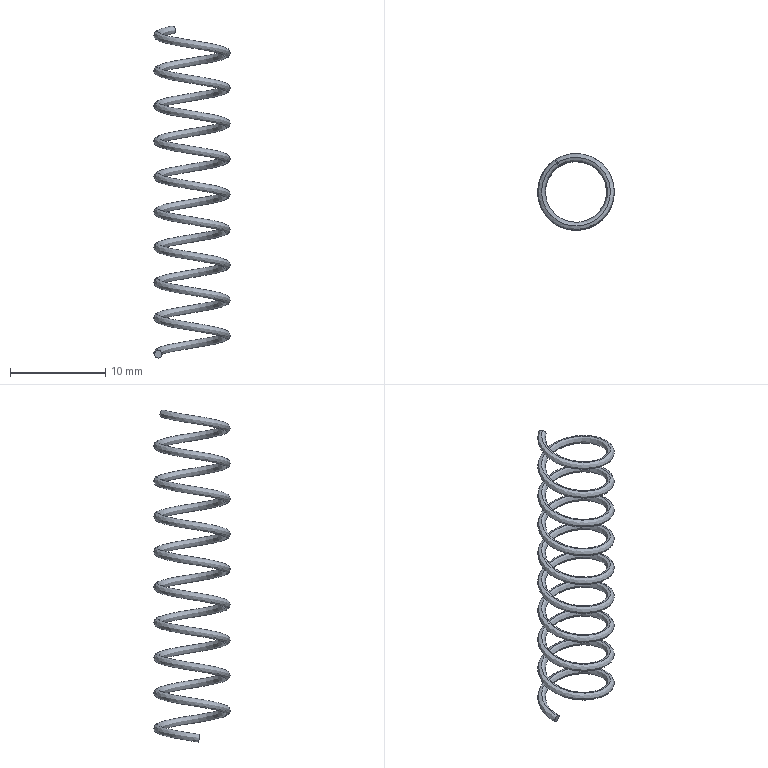Component | SolidWorks | LeftDoorAssembly-1_Spring-1 | 1 solid | 4 faces | volume 106 mm3 | spline 2 | plane 2